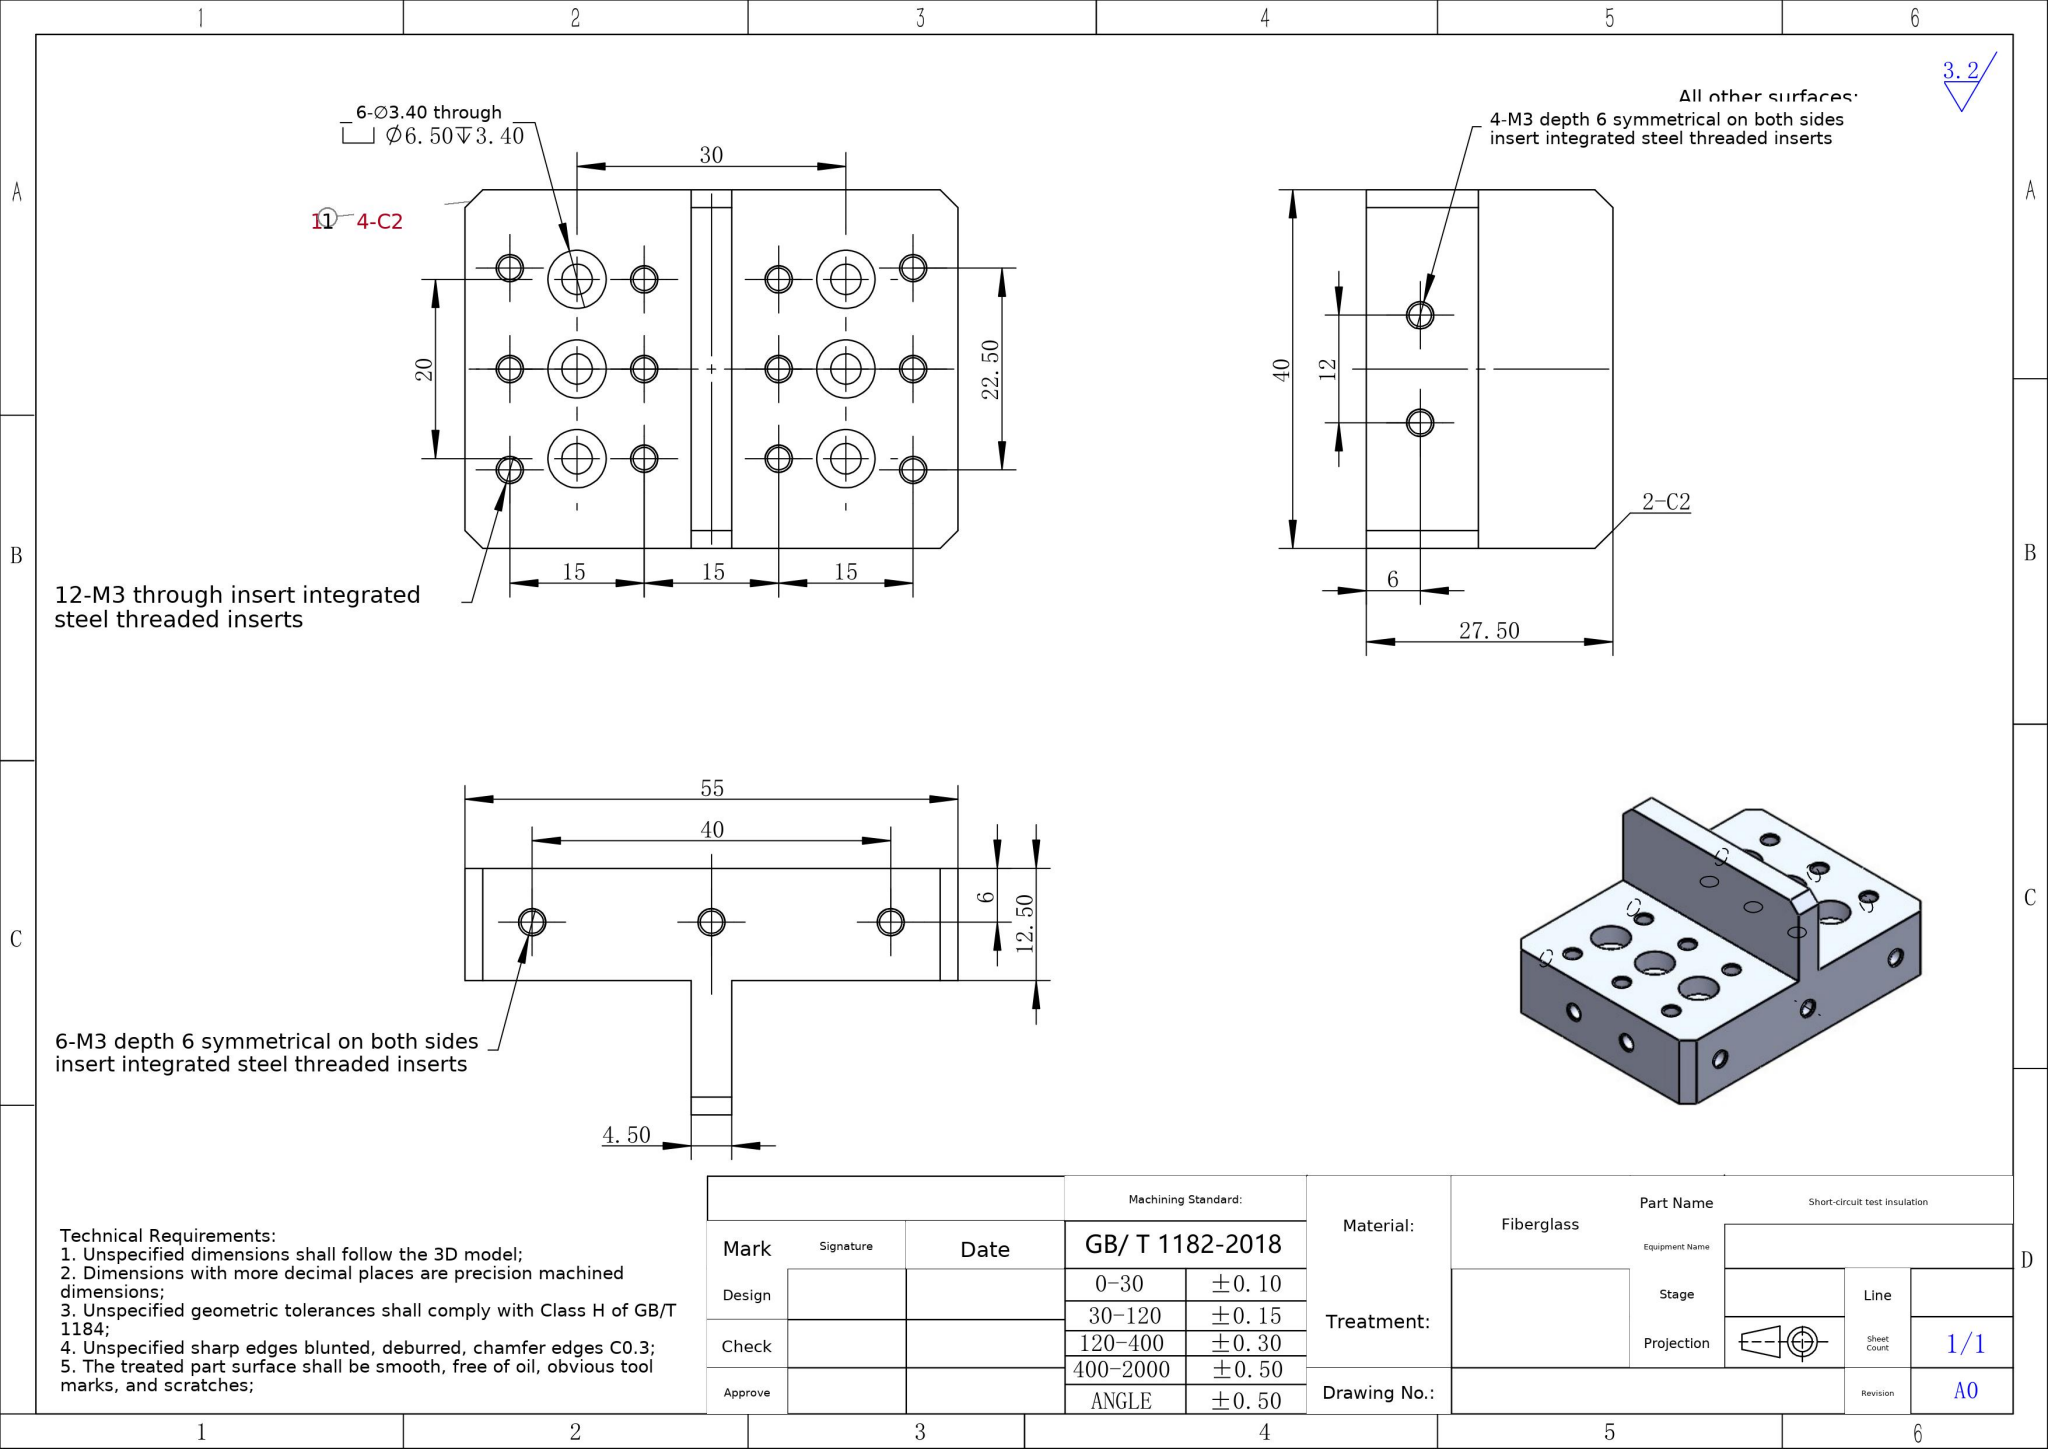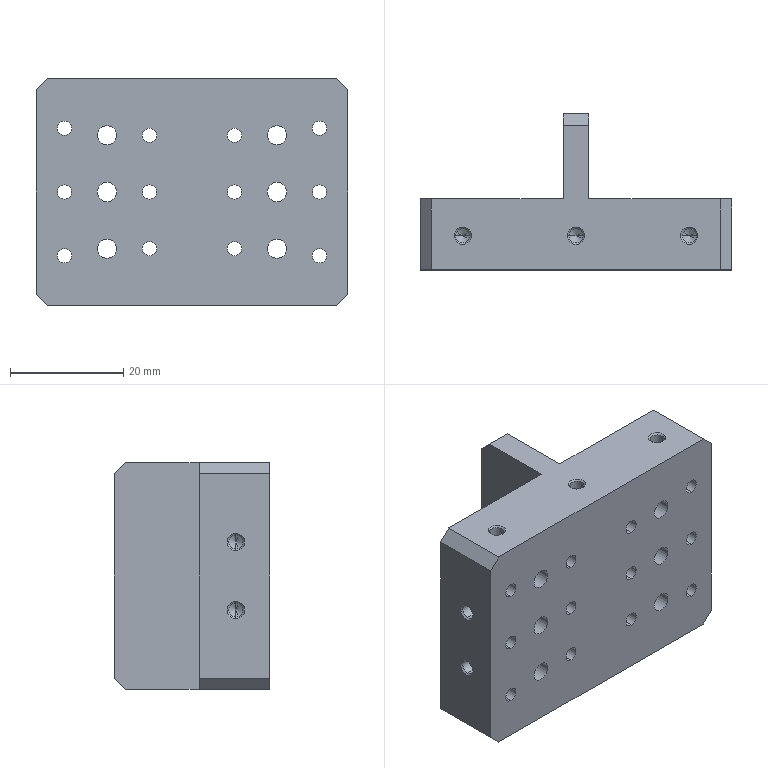Part | SolidWorks | mm | material Fiberglass | 1 solid | 154 faces | box 55 x 27.5 x 40 mm | volume 27736 mm3 | cylinder 68 | cone 64 | plane 22 | commonest cylinder face diameters 2.5 x44 6.5 x12 3.4 x12
build123d program:
from build123d import *

# Parameters (mm, degrees)
BOSS_EXTRUDE1_DEPTH         = 20
CHAMFER1_SIZE               = 2
CHAMFER2_SIZE               = 2
M3_TAPPED_HOLE4_AT_2_COUNT  = 2
M3_TAPPED_HOLE4_AT_2_PITCH  = 20
M3_TAPPED_HOLE4_AT_3_COUNT  = 2
M3_TAPPED_HOLE4_AT_3_PITCH  = 40
M3_TAPPED_HOLE6_AT_2_COUNT  = 2
M3_TAPPED_HOLE6_AT_2_PITCH  = 12
SKETCH6_R                   = 1.7
CUT_EXTRUDE1_DEPTH          = 40
SKETCH7_R                   = 3.25
CUT_EXTRUDE2_DEPTH          = 3.4
M3_TAPPED_HOLE8_D           = 2.5
M3_TAPPED_HOLE8_CSINK_D     = 3.05
M3_TAPPED_HOLE8_CSINK_ANGLE = 90


with BuildPart() as part:
    # Sketch1 → Boss-Extrude1 (new, symmetric)
    with BuildSketch(Plane.XY):
        Polygon((-27.5, 0), (27.5, 0), (27.5, 12.5), (2.25, 12.5), (2.25, 27.5), (-2.25, 27.5), (-2.25, 12.5), (-27.5, 12.5), align=None)
    extrude(amount=BOSS_EXTRUDE1_DEPTH, both=True)

    # Chamfer1
    chamfer1_edges = [part.edges().sort_by_distance(p)[0] for p in [
        (27.5, 6.25, -20),
        (-27.5, 6.25, -20),
        (27.5, 6.25, 20),
        (-27.5, 6.25, 20),
    ]]
    chamfer(chamfer1_edges, length=CHAMFER1_SIZE)

    # Chamfer2
    chamfer2_edges = [part.edges().sort_by_distance(p)[0] for p in [
        (0, 27.5, 20),
        (0, 27.5, -20),
    ]]
    chamfer(chamfer2_edges, length=CHAMFER2_SIZE)

    # Sketch3 → M3 Tapped Hole4 (revolve, cut)
    with BuildSketch(Plane(origin=(-20, 6, 20), x_dir=(0, -1, 0), z_dir=(1, 0, 0))):
        Polygon((0, 0), (0, 9.251), (1.25, 8.5), (1.25, 0.275), (1.525, 0), align=None)
    m3_tapped_hole4 = revolve(axis=Axis((-20, 6, 26.35), (0, 0, -1)), mode=Mode.SUBTRACT)

    # M3 Tapped Hole4 at 2: M3 Tapped Hole4 ×2
    with Locations(*[(i * M3_TAPPED_HOLE4_AT_2_PITCH, 0, 0) for i in range(1, M3_TAPPED_HOLE4_AT_2_COUNT)]):
        add(m3_tapped_hole4, mode=Mode.SUBTRACT)

    # M3 Tapped Hole4 at 3: M3 Tapped Hole4 ×2
    with Locations(*[(i * M3_TAPPED_HOLE4_AT_3_PITCH, 0, 0) for i in range(1, M3_TAPPED_HOLE4_AT_3_COUNT)]):
        add(m3_tapped_hole4, mode=Mode.SUBTRACT)

    # Mirror1: M3 Tapped Hole4 across plane
    add(m3_tapped_hole4.mirror(Plane.XY), mode=Mode.SUBTRACT)

    # Mirror1 copy 1 sketch → Mirror1 copy 1 (revolve, cut)
    with BuildSketch(Plane(origin=(0, 6, -20), x_dir=(0, -1, 0), z_dir=(1, 0, 0))):
        Polygon((0, 0), (0, -9.251), (1.25, -8.5), (1.25, -0.275), (1.525, 0), align=None)
    revolve(axis=Axis((0, 6, -26.35), (0, 0, -1)), mode=Mode.SUBTRACT)

    # Mirror1 copy 2 sketch → Mirror1 copy 2 (revolve, cut)
    with BuildSketch(Plane(origin=(20, 6, -20), x_dir=(0, -1, 0), z_dir=(1, 0, 0))):
        Polygon((0, 0), (0, -9.251), (1.25, -8.5), (1.25, -0.275), (1.525, 0), align=None)
    revolve(axis=Axis((20, 6, -26.35), (0, 0, -1)), mode=Mode.SUBTRACT)

    # Sketch5 → M3 Tapped Hole6 (revolve, cut)
    with BuildSketch(Plane(origin=(-27.5, 6, -6), x_dir=(0, 0, 1), z_dir=(0, 1, 0))):
        Polygon((0, 0), (0, 9.251), (1.25, 8.5), (1.25, 0.275), (1.525, 0), align=None)
    m3_tapped_hole6 = revolve(axis=Axis((-33.85, 6, -6), (1, 0, 0)), mode=Mode.SUBTRACT)

    # M3 Tapped Hole6 at 2: M3 Tapped Hole6 ×2
    with Locations(*[(0, 0, i * M3_TAPPED_HOLE6_AT_2_PITCH) for i in range(1, M3_TAPPED_HOLE6_AT_2_COUNT)]):
        add(m3_tapped_hole6, mode=Mode.SUBTRACT)

    # Mirror2: M3 Tapped Hole6 across plane
    add(m3_tapped_hole6.mirror(Plane(origin=(0, 0, 0), x_dir=(0, 0, 1), z_dir=(1, 0, 0))), mode=Mode.SUBTRACT)

    # Mirror2 copy 1 sketch → Mirror2 copy 1 (revolve, cut)
    with BuildSketch(Plane(origin=(27.5, 6, 6), x_dir=(0, 0, 1), z_dir=(0, 1, 0))):
        Polygon((0, 0), (0, -9.251), (1.25, -8.5), (1.25, -0.275), (1.525, 0), align=None)
    revolve(axis=Axis((33.85, 6, 6), (1, 0, 0)), mode=Mode.SUBTRACT)

    # Sketch6 → Cut-Extrude1 (cut)
    with BuildSketch(Plane(origin=(0, 12.5, 0), x_dir=(1, 0, 0), z_dir=(0, 1, 0))):
        with Locations(Location((15, 0, 0), (0, 0, 180))):
            Circle(SKETCH6_R)
        with Locations(Location((15, -10, 0), (0, 0, 180))):
            Circle(SKETCH6_R)
        with Locations(Location((15, 10, 0), (0, 0, 180))):
            Circle(SKETCH6_R)
        with Locations(Location((-15, -10, 0), (0, 0, 270))):
            Circle(SKETCH6_R)
        with Locations(Location((-15, 0, 0), (0, 0, 270))):
            Circle(SKETCH6_R)
        with Locations(Location((-15, 10, 0), (0, 0, 270))):
            Circle(SKETCH6_R)
    extrude(amount=-CUT_EXTRUDE1_DEPTH, mode=Mode.SUBTRACT)

    # Sketch7 → Cut-Extrude2 (cut)
    with BuildSketch(Plane(origin=(0, 12.5, 0), x_dir=(1, 0, 0), z_dir=(0, 1, 0))):
        with Locations(Location((-15, 10, 0), (0, 0, 180))):
            Circle(SKETCH7_R)
        with Locations(Location((-15, 0, 0), (0, 0, 180))):
            Circle(SKETCH7_R)
        with Locations(Location((-15, -10, 0), (0, 0, 180))):
            Circle(SKETCH7_R)
        with Locations(Location((15, 10, 0), (0, 0, 180))):
            Circle(SKETCH7_R)
        with Locations(Location((15, 0, 0), (0, 0, 180))):
            Circle(SKETCH7_R)
        with Locations(Location((15, -10, 0), (0, 0, 180))):
            Circle(SKETCH7_R)
    extrude(amount=-CUT_EXTRUDE2_DEPTH, mode=Mode.SUBTRACT)

    # M3 Tapped Hole8 (through all)
    with Locations(Plane(origin=(0, 12.5, 0), x_dir=(1, 0, 0), z_dir=(0, 1, 0))):
        with Locations((-7.5, 0), (7.5, 10), (22.5, 11.25), (22.5, -11.25), (7.5, -10), (-7.5, -10), (-22.5, -11.25), (-22.5, 11.25), (-7.5, 10), (22.5, 0), (-22.5, 0), (7.5, 0)):
            CounterSinkHole(M3_TAPPED_HOLE8_D / 2, M3_TAPPED_HOLE8_CSINK_D / 2, counter_sink_angle=M3_TAPPED_HOLE8_CSINK_ANGLE)


solid = part.part